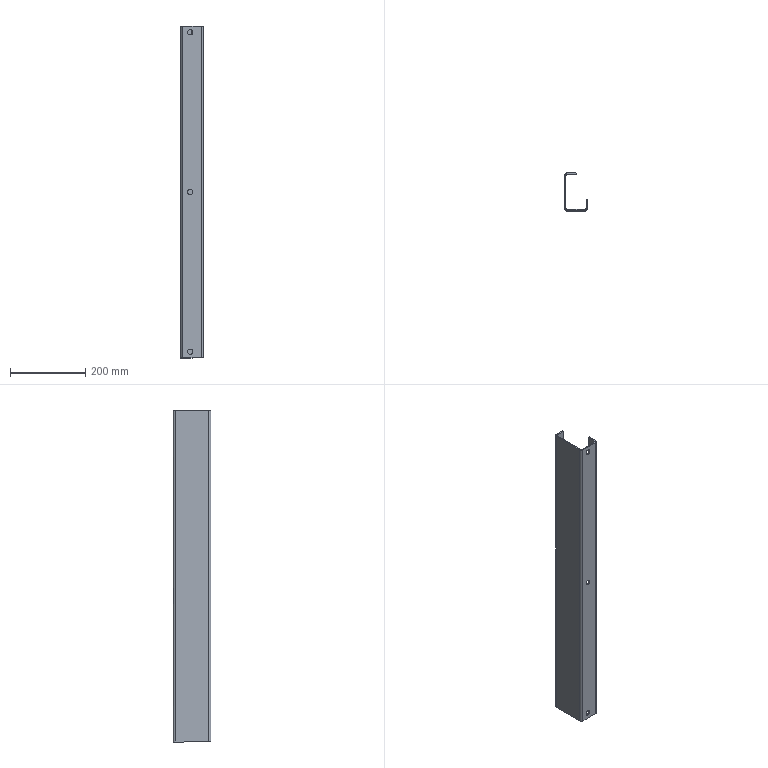Component | SolidWorks | BottomBeamAssembly-1_BottomBeam-1 | 1 solid | 50 faces | volume 538946 mm3 | plane 30 | cylinder 20 | commonest cylinder face diameters 11 x8 14 x6 6 x3 12 x3